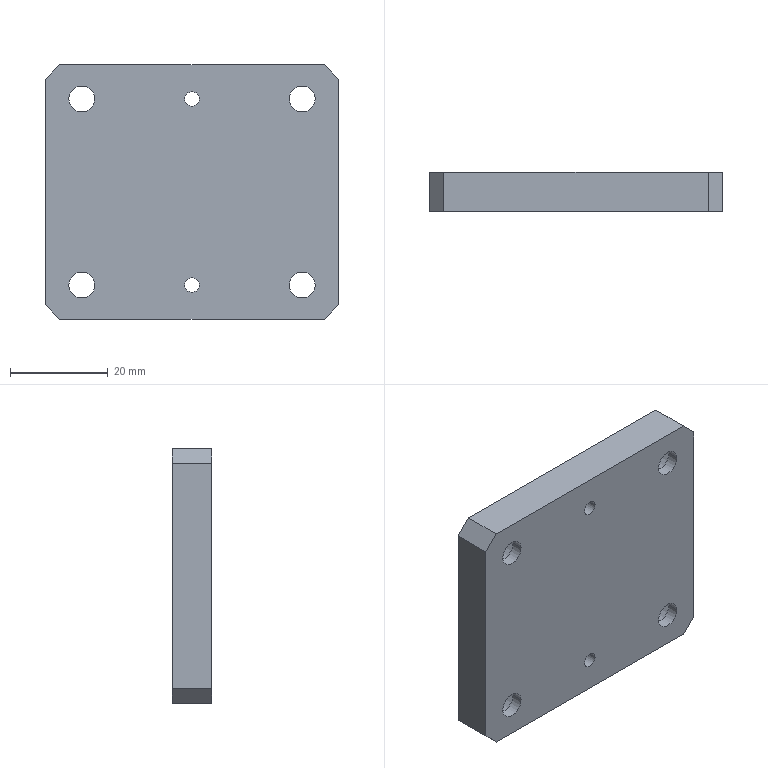Component | SolidWorks | SFTJ-08-ModuleAdapterBlock-1 | 1 solid | 34 faces | box 60 x 8 x 52 mm | volume 22709 mm3 | cylinder 20 | plane 14 | commonest cylinder face diameters 10 x8 5.3 x8 3 x4
build123d program:
from build123d import *

# Parameters (mm, degrees)
SKETCH1_W                                            = 60
SKETCH1_H                                            = 52
BOSS_EXTRUDE1_DEPTH                                  = 4
HOLE_SIZE_ACCORDING_TO_HEX_SOCKET_HEAD_C_D           = 5.3
HOLE_SIZE_ACCORDING_TO_HEX_SOCKET_HEAD_C_CBORE_D     = 10
HOLE_SIZE_ACCORDING_TO_HEX_SOCKET_HEAD_C_CBORE_DEPTH = 5.7
SIZE_MM_DOWEL_PIN_HOLE1_D                            = 3
CHAMFER1_SIZE                                        = 3


with BuildPart() as part:
    # Sketch1 → Boss-Extrude1 (new, symmetric)
    with BuildSketch(Plane.XY):
        Rectangle(SKETCH1_W, SKETCH1_H)
    extrude(amount=BOSS_EXTRUDE1_DEPTH, both=True)

    # Hole Size according to Hex Socket Head C (through all)
    with Locations(Plane.XY.offset(4)):
        with Locations((-22.5, 19), (22.5, 19), (-22.5, -19), (22.5, -19)):
            CounterBoreHole(HOLE_SIZE_ACCORDING_TO_HEX_SOCKET_HEAD_C_D / 2, HOLE_SIZE_ACCORDING_TO_HEX_SOCKET_HEAD_C_CBORE_D / 2, HOLE_SIZE_ACCORDING_TO_HEX_SOCKET_HEAD_C_CBORE_DEPTH)

    # Size mm Dowel Pin Hole1 (through all)
    with Locations(Plane(origin=(0, 0, -4), x_dir=(-1, 0, 0), z_dir=(0, 0, -1))):
        with Locations((0, -19), (0, 19)):
            Hole(SIZE_MM_DOWEL_PIN_HOLE1_D / 2)

    # Chamfer1
    chamfer1_edges = [part.edges().sort_by_distance(p)[0] for p in [
        (30, -26, 0),
        (-30, -26, 0),
        (-30, 26, 0),
        (30, 26, 0),
    ]]
    chamfer(chamfer1_edges, length=CHAMFER1_SIZE)


solid = part.part

# Placed as in the assembly
solid = solid.moved(Location((-235.009, 44.721, 38.589), (-90, 0, 0)))
STEP:
#1=COLOUR_RGB('',0.7922,0.8196,0.9333);
#2=FILL_AREA_STYLE_COLOUR('',#1);
#3=FILL_AREA_STYLE('',(#2));
#4=SURFACE_STYLE_FILL_AREA(#3);
#5=SURFACE_SIDE_STYLE('',(#4));
#6=SURFACE_STYLE_USAGE(.BOTH.,#5);
#7=PRESENTATION_STYLE_ASSIGNMENT((#6));
#8=CARTESIAN_POINT('',(-9.193,1.918,2.267));
#9=VERTEX_POINT('',#8);
#10=CARTESIAN_POINT('',(-9.311,1.918,2.267));
#11=VERTEX_POINT('',#10);
#12=CARTESIAN_POINT('',(-9.252,1.918,2.267));
#13=DIRECTION('',(0.,-1.,-0.));
#14=DIRECTION('',(-1.,0.,0.));
#15=AXIS2_PLACEMENT_3D('',#12,#13,#14);
#16=CIRCLE('',#15,0.05906);
#17=EDGE_CURVE('',#9,#11,#16,.T.);
#18=ORIENTED_EDGE('',*,*,#17,.F.);
#19=CARTESIAN_POINT('',(-9.193,1.603,2.267));
#20=VERTEX_POINT('',#19);
#21=CARTESIAN_POINT('',(-9.193,1.603,2.267));
#22=DIRECTION('',(0.,-1.,-0.));
#23=VECTOR('',#22,39.37);
#24=LINE('',#21,#23);
#25=EDGE_CURVE('',#9,#20,#24,.T.);
#26=ORIENTED_EDGE('',*,*,#25,.T.);
#27=CARTESIAN_POINT('',(-9.311,1.603,2.267));
#28=VERTEX_POINT('',#27);
#29=CARTESIAN_POINT('',(-9.252,1.603,2.267));
#30=DIRECTION('',(0.,-1.,-0.));
#31=DIRECTION('',(-1.,0.,0.));
#32=AXIS2_PLACEMENT_3D('',#29,#30,#31);
#33=CIRCLE('',#32,0.05906);
#34=EDGE_CURVE('',#20,#28,#33,.T.);
#35=ORIENTED_EDGE('',*,*,#34,.T.);
#36=CARTESIAN_POINT('',(-9.311,1.603,2.267));
#37=DIRECTION('',(0.,-1.,-0.));
#38=VECTOR('',#37,39.37);
#39=LINE('',#36,#38);
#40=EDGE_CURVE('',#11,#28,#39,.T.);
#41=ORIENTED_EDGE('',*,*,#40,.F.);
#42=EDGE_LOOP('',(#18,#26,#35,#41));
#43=FACE_OUTER_BOUND('',#42,.T.);
#44=CARTESIAN_POINT('',(-9.252,1.603,2.267));
#45=DIRECTION('',(0.,-1.,-0.));
#46=DIRECTION('',(-1.,0.,0.));
#47=AXIS2_PLACEMENT_3D('',#44,#45,#46);
#48=CYLINDRICAL_SURFACE('',#47,0.05906);
#49=ADVANCED_FACE('',(#43),#48,.F.);
#50=CARTESIAN_POINT('',(-9.193,1.918,0.7712));
#51=VERTEX_POINT('',#50);
#52=CARTESIAN_POINT('',(-9.311,1.918,0.7712));
#53=VERTEX_POINT('',#52);
#54=CARTESIAN_POINT('',(-9.252,1.918,0.7712));
#55=DIRECTION('',(0.,-1.,-0.));
#56=DIRECTION('',(-1.,0.,0.));
#57=AXIS2_PLACEMENT_3D('',#54,#55,#56);
#58=CIRCLE('',#57,0.05906);
#59=EDGE_CURVE('',#51,#53,#58,.T.);
#60=ORIENTED_EDGE('',*,*,#59,.F.);
#61=CARTESIAN_POINT('',(-9.193,1.603,0.7712));
#62=VERTEX_POINT('',#61);
#63=CARTESIAN_POINT('',(-9.193,1.603,0.7712));
#64=DIRECTION('',(0.,-1.,-0.));
#65=VECTOR('',#64,39.37);
#66=LINE('',#63,#65);
#67=EDGE_CURVE('',#51,#62,#66,.T.);
#68=ORIENTED_EDGE('',*,*,#67,.T.);
#69=CARTESIAN_POINT('',(-9.311,1.603,0.7712));
#70=VERTEX_POINT('',#69);
#71=CARTESIAN_POINT('',(-9.252,1.603,0.7712));
#72=DIRECTION('',(0.,-1.,-0.));
#73=DIRECTION('',(-1.,0.,0.));
#74=AXIS2_PLACEMENT_3D('',#71,#72,#73);
#75=CIRCLE('',#74,0.05906);
#76=EDGE_CURVE('',#62,#70,#75,.T.);
#77=ORIENTED_EDGE('',*,*,#76,.T.);
#78=CARTESIAN_POINT('',(-9.311,1.603,0.7712));
#79=DIRECTION('',(0.,-1.,-0.));
#80=VECTOR('',#79,39.37);
#81=LINE('',#78,#80);
#82=EDGE_CURVE('',#53,#70,#81,.T.);
#83=ORIENTED_EDGE('',*,*,#82,.F.);
#84=EDGE_LOOP('',(#60,#68,#77,#83));
#85=FACE_OUTER_BOUND('',#84,.T.);
#86=CARTESIAN_POINT('',(-9.252,1.603,0.7712));
#87=DIRECTION('',(0.,-1.,-0.));
#88=DIRECTION('',(-1.,0.,0.));
#89=AXIS2_PLACEMENT_3D('',#86,#87,#88);
#90=CYLINDRICAL_SURFACE('',#89,0.05906);
#91=ADVANCED_FACE('',(#85),#90,.F.);
#92=CARTESIAN_POINT('',(-10.335,1.694,0.7712));
#93=VERTEX_POINT('',#92);
#94=CARTESIAN_POINT('',(-9.941,1.694,0.7712));
#95=VERTEX_POINT('',#94);
#96=CARTESIAN_POINT('',(-10.138,1.694,0.7712));
#97=DIRECTION('',(-0.,1.,0.));
#98=DIRECTION('',(1.,0.,0.));
#99=AXIS2_PLACEMENT_3D('',#96,#97,#98);
#100=CIRCLE('',#99,0.1969);
#101=EDGE_CURVE('',#93,#95,#100,.T.);
#102=ORIENTED_EDGE('',*,*,#101,.F.);
#103=CARTESIAN_POINT('',(-10.335,1.918,0.7712));
#104=VERTEX_POINT('',#103);
#105=CARTESIAN_POINT('',(-10.335,1.918,0.7712));
#106=DIRECTION('',(-0.,1.,0.));
#107=VECTOR('',#106,39.37);
#108=LINE('',#105,#107);
#109=EDGE_CURVE('',#93,#104,#108,.T.);
#110=ORIENTED_EDGE('',*,*,#109,.T.);
#111=CARTESIAN_POINT('',(-9.941,1.918,0.7712));
#112=VERTEX_POINT('',#111);
#113=CARTESIAN_POINT('',(-10.138,1.918,0.7712));
#114=DIRECTION('',(-0.,1.,0.));
#115=DIRECTION('',(1.,0.,0.));
#116=AXIS2_PLACEMENT_3D('',#113,#114,#115);
#117=CIRCLE('',#116,0.1969);
#118=EDGE_CURVE('',#104,#112,#117,.T.);
#119=ORIENTED_EDGE('',*,*,#118,.T.);
#120=CARTESIAN_POINT('',(-9.941,1.918,0.7712));
#121=DIRECTION('',(-0.,1.,0.));
#122=VECTOR('',#121,39.37);
#123=LINE('',#120,#122);
#124=EDGE_CURVE('',#95,#112,#123,.T.);
#125=ORIENTED_EDGE('',*,*,#124,.F.);
#126=EDGE_LOOP('',(#102,#110,#119,#125));
#127=FACE_OUTER_BOUND('',#126,.T.);
#128=CARTESIAN_POINT('',(-10.138,1.918,0.7712));
#129=DIRECTION('',(-0.,1.,0.));
#130=DIRECTION('',(1.,0.,0.));
#131=AXIS2_PLACEMENT_3D('',#128,#129,#130);
#132=CYLINDRICAL_SURFACE('',#131,0.1969);
#133=ADVANCED_FACE('',(#127),#132,.F.);
#134=CARTESIAN_POINT('',(-10.242,1.603,0.7712));
#135=VERTEX_POINT('',#134);
#136=CARTESIAN_POINT('',(-10.034,1.603,0.7712));
#137=VERTEX_POINT('',#136);
#138=CARTESIAN_POINT('',(-10.138,1.603,0.7712));
#139=DIRECTION('',(-0.,1.,0.));
#140=DIRECTION('',(1.,0.,0.));
#141=AXIS2_PLACEMENT_3D('',#138,#139,#140);
#142=CIRCLE('',#141,0.1043);
#143=EDGE_CURVE('',#135,#137,#142,.T.);
#144=ORIENTED_EDGE('',*,*,#143,.F.);
#145=CARTESIAN_POINT('',(-10.242,1.694,0.7712));
#146=VERTEX_POINT('',#145);
#147=CARTESIAN_POINT('',(-10.242,1.918,0.7712));
#148=DIRECTION('',(-0.,1.,0.));
#149=VECTOR('',#148,39.37);
#150=LINE('',#147,#149);
#151=EDGE_CURVE('',#135,#146,#150,.T.);
#152=ORIENTED_EDGE('',*,*,#151,.T.);
#153=CARTESIAN_POINT('',(-10.034,1.694,0.7712));
#154=VERTEX_POINT('',#153);
#155=CARTESIAN_POINT('',(-10.138,1.694,0.7712));
#156=DIRECTION('',(-0.,1.,0.));
#157=DIRECTION('',(1.,0.,0.));
#158=AXIS2_PLACEMENT_3D('',#155,#156,#157);
#159=CIRCLE('',#158,0.1043);
#160=EDGE_CURVE('',#146,#154,#159,.T.);
#161=ORIENTED_EDGE('',*,*,#160,.T.);
#162=CARTESIAN_POINT('',(-10.034,1.918,0.7712));
#163=DIRECTION('',(-0.,1.,0.));
#164=VECTOR('',#163,39.37);
#165=LINE('',#162,#164);
#166=EDGE_CURVE('',#137,#154,#165,.T.);
#167=ORIENTED_EDGE('',*,*,#166,.F.);
#168=EDGE_LOOP('',(#144,#152,#161,#167));
#169=FACE_OUTER_BOUND('',#168,.T.);
#170=CARTESIAN_POINT('',(-10.138,1.918,0.7712));
#171=DIRECTION('',(-0.,1.,0.));
#172=DIRECTION('',(1.,0.,0.));
#173=AXIS2_PLACEMENT_3D('',#170,#171,#172);
#174=CYLINDRICAL_SURFACE('',#173,0.1043);
#175=ADVANCED_FACE('',(#169),#174,.F.);
#176=CARTESIAN_POINT('',(-8.563,1.694,0.7712));
#177=VERTEX_POINT('',#176);
#178=CARTESIAN_POINT('',(-8.17,1.694,0.7712));
#179=VERTEX_POINT('',#178);
#180=CARTESIAN_POINT('',(-8.367,1.694,0.7712));
#181=DIRECTION('',(-0.,1.,0.));
#182=DIRECTION('',(1.,0.,0.));
#183=AXIS2_PLACEMENT_3D('',#180,#181,#182);
#184=CIRCLE('',#183,0.1969);
#185=EDGE_CURVE('',#177,#179,#184,.T.);
#186=ORIENTED_EDGE('',*,*,#185,.F.);
#187=CARTESIAN_POINT('',(-8.563,1.918,0.7712));
#188=VERTEX_POINT('',#187);
#189=CARTESIAN_POINT('',(-8.563,1.918,0.7712));
#190=DIRECTION('',(-0.,1.,0.));
#191=VECTOR('',#190,39.37);
#192=LINE('',#189,#191);
#193=EDGE_CURVE('',#177,#188,#192,.T.);
#194=ORIENTED_EDGE('',*,*,#193,.T.);
#195=CARTESIAN_POINT('',(-8.17,1.918,0.7712));
#196=VERTEX_POINT('',#195);
#197=CARTESIAN_POINT('',(-8.367,1.918,0.7712));
#198=DIRECTION('',(-0.,1.,0.));
#199=DIRECTION('',(1.,0.,0.));
#200=AXIS2_PLACEMENT_3D('',#197,#198,#199);
#201=CIRCLE('',#200,0.1969);
#202=EDGE_CURVE('',#188,#196,#201,.T.);
#203=ORIENTED_EDGE('',*,*,#202,.T.);
#204=CARTESIAN_POINT('',(-8.17,1.918,0.7712));
#205=DIRECTION('',(-0.,1.,0.));
#206=VECTOR('',#205,39.37);
#207=LINE('',#204,#206);
#208=EDGE_CURVE('',#179,#196,#207,.T.);
#209=ORIENTED_EDGE('',*,*,#208,.F.);
#210=EDGE_LOOP('',(#186,#194,#203,#209));
#211=FACE_OUTER_BOUND('',#210,.T.);
#212=CARTESIAN_POINT('',(-8.367,1.918,0.7712));
#213=DIRECTION('',(-0.,1.,0.));
#214=DIRECTION('',(1.,0.,0.));
#215=AXIS2_PLACEMENT_3D('',#212,#213,#214);
#216=CYLINDRICAL_SURFACE('',#215,0.1969);
#217=ADVANCED_FACE('',(#211),#216,.F.);
#218=CARTESIAN_POINT('',(-8.471,1.603,0.7712));
#219=VERTEX_POINT('',#218);
#220=CARTESIAN_POINT('',(-8.262,1.603,0.7712));
#221=VERTEX_POINT('',#220);
#222=CARTESIAN_POINT('',(-8.367,1.603,0.7712));
#223=DIRECTION('',(-0.,1.,0.));
#224=DIRECTION('',(1.,0.,0.));
#225=AXIS2_PLACEMENT_3D('',#222,#223,#224);
#226=CIRCLE('',#225,0.1043);
#227=EDGE_CURVE('',#219,#221,#226,.T.);
#228=ORIENTED_EDGE('',*,*,#227,.F.);
#229=CARTESIAN_POINT('',(-8.471,1.694,0.7712));
#230=VERTEX_POINT('',#229);
#231=CARTESIAN_POINT('',(-8.471,1.918,0.7712));
#232=DIRECTION('',(-0.,1.,0.));
#233=VECTOR('',#232,39.37);
#234=LINE('',#231,#233);
#235=EDGE_CURVE('',#219,#230,#234,.T.);
#236=ORIENTED_EDGE('',*,*,#235,.T.);
#237=CARTESIAN_POINT('',(-8.262,1.694,0.7712));
#238=VERTEX_POINT('',#237);
#239=CARTESIAN_POINT('',(-8.367,1.694,0.7712));
#240=DIRECTION('',(-0.,1.,0.));
#241=DIRECTION('',(1.,0.,0.));
#242=AXIS2_PLACEMENT_3D('',#239,#240,#241);
#243=CIRCLE('',#242,0.1043);
#244=EDGE_CURVE('',#230,#238,#243,.T.);
#245=ORIENTED_EDGE('',*,*,#244,.T.);
#246=CARTESIAN_POINT('',(-8.262,1.918,0.7712));
#247=DIRECTION('',(-0.,1.,0.));
#248=VECTOR('',#247,39.37);
#249=LINE('',#246,#248);
#250=EDGE_CURVE('',#221,#238,#249,.T.);
#251=ORIENTED_EDGE('',*,*,#250,.F.);
#252=EDGE_LOOP('',(#228,#236,#245,#251));
#253=FACE_OUTER_BOUND('',#252,.T.);
#254=CARTESIAN_POINT('',(-8.367,1.918,0.7712));
#255=DIRECTION('',(-0.,1.,0.));
#256=DIRECTION('',(1.,0.,0.));
#257=AXIS2_PLACEMENT_3D('',#254,#255,#256);
#258=CYLINDRICAL_SURFACE('',#257,0.1043);
#259=ADVANCED_FACE('',(#253),#258,.F.);
#260=CARTESIAN_POINT('',(-10.335,1.694,2.267));
#261=VERTEX_POINT('',#260);
#262=CARTESIAN_POINT('',(-9.941,1.694,2.267));
#263=VERTEX_POINT('',#262);
#264=CARTESIAN_POINT('',(-10.138,1.694,2.267));
#265=DIRECTION('',(-0.,1.,0.));
#266=DIRECTION('',(1.,0.,0.));
#267=AXIS2_PLACEMENT_3D('',#264,#265,#266);
#268=CIRCLE('',#267,0.1969);
#269=EDGE_CURVE('',#261,#263,#268,.T.);
#270=ORIENTED_EDGE('',*,*,#269,.F.);
#271=CARTESIAN_POINT('',(-10.335,1.918,2.267));
#272=VERTEX_POINT('',#271);
#273=CARTESIAN_POINT('',(-10.335,1.918,2.267));
#274=DIRECTION('',(-0.,1.,0.));
#275=VECTOR('',#274,39.37);
#276=LINE('',#273,#275);
#277=EDGE_CURVE('',#261,#272,#276,.T.);
#278=ORIENTED_EDGE('',*,*,#277,.T.);
#279=CARTESIAN_POINT('',(-9.941,1.918,2.267));
#280=VERTEX_POINT('',#279);
#281=CARTESIAN_POINT('',(-10.138,1.918,2.267));
#282=DIRECTION('',(-0.,1.,0.));
#283=DIRECTION('',(1.,0.,0.));
#284=AXIS2_PLACEMENT_3D('',#281,#282,#283);
#285=CIRCLE('',#284,0.1969);
#286=EDGE_CURVE('',#272,#280,#285,.T.);
#287=ORIENTED_EDGE('',*,*,#286,.T.);
#288=CARTESIAN_POINT('',(-9.941,1.918,2.267));
#289=DIRECTION('',(-0.,1.,0.));
#290=VECTOR('',#289,39.37);
#291=LINE('',#288,#290);
#292=EDGE_CURVE('',#263,#280,#291,.T.);
#293=ORIENTED_EDGE('',*,*,#292,.F.);
#294=EDGE_LOOP('',(#270,#278,#287,#293));
#295=FACE_OUTER_BOUND('',#294,.T.);
#296=CARTESIAN_POINT('',(-10.138,1.918,2.267));
#297=DIRECTION('',(-0.,1.,0.));
#298=DIRECTION('',(1.,0.,0.));
#299=AXIS2_PLACEMENT_3D('',#296,#297,#298);
#300=CYLINDRICAL_SURFACE('',#299,0.1969);
#301=ADVANCED_FACE('',(#295),#300,.F.);
#302=CARTESIAN_POINT('',(-10.242,1.603,2.267));
#303=VERTEX_POINT('',#302);
#304=CARTESIAN_POINT('',(-10.034,1.603,2.267));
#305=VERTEX_POINT('',#304);
#306=CARTESIAN_POINT('',(-10.138,1.603,2.267));
#307=DIRECTION('',(-0.,1.,0.));
#308=DIRECTION('',(1.,0.,0.));
#309=AXIS2_PLACEMENT_3D('',#306,#307,#308);
#310=CIRCLE('',#309,0.1043);
#311=EDGE_CURVE('',#303,#305,#310,.T.);
#312=ORIENTED_EDGE('',*,*,#311,.F.);
#313=CARTESIAN_POINT('',(-10.242,1.694,2.267));
#314=VERTEX_POINT('',#313);
#315=CARTESIAN_POINT('',(-10.242,1.918,2.267));
#316=DIRECTION('',(-0.,1.,0.));
#317=VECTOR('',#316,39.37);
#318=LINE('',#315,#317);
#319=EDGE_CURVE('',#303,#314,#318,.T.);
#320=ORIENTED_EDGE('',*,*,#319,.T.);
#321=CARTESIAN_POINT('',(-10.034,1.694,2.267));
#322=VERTEX_POINT('',#321);
#323=CARTESIAN_POINT('',(-10.138,1.694,2.267));
#324=DIRECTION('',(-0.,1.,0.));
#325=DIRECTION('',(1.,0.,0.));
#326=AXIS2_PLACEMENT_3D('',#323,#324,#325);
#327=CIRCLE('',#326,0.1043);
#328=EDGE_CURVE('',#314,#322,#327,.T.);
#329=ORIENTED_EDGE('',*,*,#328,.T.);
#330=CARTESIAN_POINT('',(-10.034,1.918,2.267));
#331=DIRECTION('',(-0.,1.,0.));
#332=VECTOR('',#331,39.37);
#333=LINE('',#330,#332);
#334=EDGE_CURVE('',#305,#322,#333,.T.);
#335=ORIENTED_EDGE('',*,*,#334,.F.);
#336=EDGE_LOOP('',(#312,#320,#329,#335));
#337=FACE_OUTER_BOUND('',#336,.T.);
#338=CARTESIAN_POINT('',(-10.138,1.918,2.267));
#339=DIRECTION('',(-0.,1.,0.));
#340=DIRECTION('',(1.,0.,0.));
#341=AXIS2_PLACEMENT_3D('',#338,#339,#340);
#342=CYLINDRICAL_SURFACE('',#341,0.1043);
#343=ADVANCED_FACE('',(#337),#342,.F.);
#344=CARTESIAN_POINT('',(-8.563,1.694,2.267));
#345=VERTEX_POINT('',#344);
#346=CARTESIAN_POINT('',(-8.17,1.694,2.267));
#347=VERTEX_POINT('',#346);
#348=CARTESIAN_POINT('',(-8.367,1.694,2.267));
#349=DIRECTION('',(-0.,1.,0.));
#350=DIRECTION('',(1.,0.,0.));
#351=AXIS2_PLACEMENT_3D('',#348,#349,#350);
#352=CIRCLE('',#351,0.1969);
#353=EDGE_CURVE('',#345,#347,#352,.T.);
#354=ORIENTED_EDGE('',*,*,#353,.F.);
#355=CARTESIAN_POINT('',(-8.563,1.918,2.267));
#356=VERTEX_POINT('',#355);
#357=CARTESIAN_POINT('',(-8.563,1.918,2.267));
#358=DIRECTION('',(-0.,1.,0.));
#359=VECTOR('',#358,39.37);
#360=LINE('',#357,#359);
#361=EDGE_CURVE('',#345,#356,#360,.T.);
#362=ORIENTED_EDGE('',*,*,#361,.T.);
#363=CARTESIAN_POINT('',(-8.17,1.918,2.267));
#364=VERTEX_POINT('',#363);
#365=CARTESIAN_POINT('',(-8.367,1.918,2.267));
#366=DIRECTION('',(-0.,1.,0.));
#367=DIRECTION('',(1.,0.,0.));
#368=AXIS2_PLACEMENT_3D('',#365,#366,#367);
#369=CIRCLE('',#368,0.1969);
#370=EDGE_CURVE('',#356,#364,#369,.T.);
#371=ORIENTED_EDGE('',*,*,#370,.T.);
#372=CARTESIAN_POINT('',(-8.17,1.918,2.267));
#373=DIRECTION('',(-0.,1.,0.));
#374=VECTOR('',#373,39.37);
#375=LINE('',#372,#374);
#376=EDGE_CURVE('',#347,#364,#375,.T.);
#377=ORIENTED_EDGE('',*,*,#376,.F.);
#378=EDGE_LOOP('',(#354,#362,#371,#377));
#379=FACE_OUTER_BOUND('',#378,.T.);
#380=CARTESIAN_POINT('',(-8.367,1.918,2.267));
#381=DIRECTION('',(-0.,1.,0.));
#382=DIRECTION('',(1.,0.,0.));
#383=AXIS2_PLACEMENT_3D('',#380,#381,#382);
#384=CYLINDRICAL_SURFACE('',#383,0.1969);
#385=ADVANCED_FACE('',(#379),#384,.F.);
#386=CARTESIAN_POINT('',(-8.471,1.603,2.267));
#387=VERTEX_POINT('',#386);
#388=CARTESIAN_POINT('',(-8.262,1.603,2.267));
#389=VERTEX_POINT('',#388);
#390=CARTESIAN_POINT('',(-8.367,1.603,2.267));
#391=DIRECTION('',(-0.,1.,0.));
#392=DIRECTION('',(1.,0.,0.));
#393=AXIS2_PLACEMENT_3D('',#390,#391,#392);
#394=CIRCLE('',#393,0.1043);
#395=EDGE_CURVE('',#387,#389,#394,.T.);
#396=ORIENTED_EDGE('',*,*,#395,.F.);
#397=CARTESIAN_POINT('',(-8.471,1.694,2.267));
#398=VERTEX_POINT('',#397);
#399=CARTESIAN_POINT('',(-8.471,1.918,2.267));
#400=DIRECTION('',(-0.,1.,0.));
#401=VECTOR('',#400,39.37);
#402=LINE('',#399,#401);
#403=EDGE_CURVE('',#387,#398,#402,.T.);
#404=ORIENTED_EDGE('',*,*,#403,.T.);
#405=CARTESIAN_POINT('',(-8.262,1.694,2.267));
#406=VERTEX_POINT('',#405);
#407=CARTESIAN_POINT('',(-8.367,1.694,2.267));
#408=DIRECTION('',(-0.,1.,0.));
#409=DIRECTION('',(1.,0.,0.));
#410=AXIS2_PLACEMENT_3D('',#407,#408,#409);
#411=CIRCLE('',#410,0.1043);
#412=EDGE_CURVE('',#398,#406,#411,.T.);
#413=ORIENTED_EDGE('',*,*,#412,.T.);
#414=CARTESIAN_POINT('',(-8.262,1.918,2.267));
#415=DIRECTION('',(-0.,1.,0.));
#416=VECTOR('',#415,39.37);
#417=LINE('',#414,#416);
#418=EDGE_CURVE('',#389,#406,#417,.T.);
#419=ORIENTED_EDGE('',*,*,#418,.F.);
#420=EDGE_LOOP('',(#396,#404,#413,#419));
#421=FACE_OUTER_BOUND('',#420,.T.);
#422=CARTESIAN_POINT('',(-8.367,1.918,2.267));
#423=DIRECTION('',(-0.,1.,0.));
#424=DIRECTION('',(1.,0.,0.));
#425=AXIS2_PLACEMENT_3D('',#422,#423,#424);
#426=CYLINDRICAL_SURFACE('',#425,0.1043);
#427=ADVANCED_FACE('',(#421),#426,.F.);
#428=CARTESIAN_POINT('',(-8.071,1.918,2.425));
#429=VERTEX_POINT('',#428);
#430=CARTESIAN_POINT('',(-8.071,1.918,0.6137));
#431=VERTEX_POINT('',#430);
#432=CARTESIAN_POINT('',(-8.071,1.918,0.4956));
#433=DIRECTION('',(-0.,0.,-1.));
#434=VECTOR('',#433,39.37);
#435=LINE('',#432,#434);
#436=EDGE_CURVE('',#429,#431,#435,.T.);
#437=ORIENTED_EDGE('',*,*,#436,.F.);
#438=CARTESIAN_POINT('',(-8.071,1.603,2.425));
#439=VERTEX_POINT('',#438);
#440=CARTESIAN_POINT('',(-8.071,1.918,2.425));
#441=DIRECTION('',(0.,-1.,-0.));
#442=VECTOR('',#441,39.37);
#443=LINE('',#440,#442);
#444=EDGE_CURVE('',#429,#439,#443,.T.);
#445=ORIENTED_EDGE('',*,*,#444,.T.);
#446=CARTESIAN_POINT('',(-8.071,1.603,0.6137));
#447=VERTEX_POINT('',#446);
#448=CARTESIAN_POINT('',(-8.071,1.603,0.4956));
#449=DIRECTION('',(-0.,0.,-1.));
#450=VECTOR('',#449,39.37);
#451=LINE('',#448,#450);
#452=EDGE_CURVE('',#439,#447,#451,.T.);
#453=ORIENTED_EDGE('',*,*,#452,.T.);
#454=CARTESIAN_POINT('',(-8.071,1.918,0.6137));
#455=DIRECTION('',(-0.,1.,0.));
#456=VECTOR('',#455,39.37);
#457=LINE('',#454,#456);
#458=EDGE_CURVE('',#447,#431,#457,.T.);
#459=ORIENTED_EDGE('',*,*,#458,.T.);
#460=EDGE_LOOP('',(#437,#445,#453,#459));
#461=FACE_OUTER_BOUND('',#460,.T.);
#462=CARTESIAN_POINT('',(-8.071,1.918,0.4956));
#463=DIRECTION('',(-1.,-0.,0.));
#464=DIRECTION('',(0.,-0.,1.));
#465=AXIS2_PLACEMENT_3D('',#462,#463,#464);
#466=PLANE('',#465);
#467=ADVANCED_FACE('',(#461),#466,.F.);
#468=CARTESIAN_POINT('',(-8.189,1.918,0.4956));
#469=VERTEX_POINT('',#468);
#470=CARTESIAN_POINT('',(-10.315,1.918,0.4956));
#471=VERTEX_POINT('',#470);
#472=CARTESIAN_POINT('',(-10.433,1.918,0.4956));
#473=DIRECTION('',(-1.,-0.,-0.));
#474=VECTOR('',#473,39.37);
#475=LINE('',#472,#474);
#476=EDGE_CURVE('',#469,#471,#475,.T.);
#477=ORIENTED_EDGE('',*,*,#476,.F.);
#478=CARTESIAN_POINT('',(-8.189,1.603,0.4956));
#479=VERTEX_POINT('',#478);
#480=CARTESIAN_POINT('',(-8.189,1.918,0.4956));
#481=DIRECTION('',(0.,-1.,-0.));
#482=VECTOR('',#481,39.37);
#483=LINE('',#480,#482);
#484=EDGE_CURVE('',#469,#479,#483,.T.);
#485=ORIENTED_EDGE('',*,*,#484,.T.);
#486=CARTESIAN_POINT('',(-10.315,1.603,0.4956));
#487=VERTEX_POINT('',#486);
#488=CARTESIAN_POINT('',(-10.433,1.603,0.4956));
#489=DIRECTION('',(-1.,-0.,-0.));
#490=VECTOR('',#489,39.37);
#491=LINE('',#488,#490);
#492=EDGE_CURVE('',#479,#487,#491,.T.);
#493=ORIENTED_EDGE('',*,*,#492,.T.);
#494=CARTESIAN_POINT('',(-10.315,1.918,0.4956));
#495=DIRECTION('',(-0.,1.,0.));
#496=VECTOR('',#495,39.37);
#497=LINE('',#494,#496);
#498=EDGE_CURVE('',#487,#471,#497,.T.);
#499=ORIENTED_EDGE('',*,*,#498,.T.);
#500=EDGE_LOOP('',(#477,#485,#493,#499));
#501=FACE_OUTER_BOUND('',#500,.T.);
#502=CARTESIAN_POINT('',(-10.433,1.918,0.4956));
#503=DIRECTION('',(-0.,-0.,1.));
#504=DIRECTION('',(0.,-1.,-0.));
#505=AXIS2_PLACEMENT_3D('',#502,#503,#504);
#506=PLANE('',#505);
#507=ADVANCED_FACE('',(#501),#506,.F.);
#508=CARTESIAN_POINT('',(-10.433,1.603,0.6137));
#509=VERTEX_POINT('',#508);
#510=CARTESIAN_POINT('',(-10.433,1.603,2.425));
#511=VERTEX_POINT('',#510);
#512=CARTESIAN_POINT('',(-10.433,1.603,0.4956));
#513=DIRECTION('',(0.,-0.,1.));
#514=VECTOR('',#513,39.37);
#515=LINE('',#512,#514);
#516=EDGE_CURVE('',#509,#511,#515,.T.);
#517=ORIENTED_EDGE('',*,*,#516,.T.);
#518=CARTESIAN_POINT('',(-10.433,1.918,2.425));
#519=VERTEX_POINT('',#518);
#520=CARTESIAN_POINT('',(-10.433,1.918,2.425));
#521=DIRECTION('',(-0.,1.,0.));
#522=VECTOR('',#521,39.37);
#523=LINE('',#520,#522);
#524=EDGE_CURVE('',#511,#519,#523,.T.);
#525=ORIENTED_EDGE('',*,*,#524,.T.);
#526=CARTESIAN_POINT('',(-10.433,1.918,0.6137));
#527=VERTEX_POINT('',#526);
#528=CARTESIAN_POINT('',(-10.433,1.918,0.4956));
#529=DIRECTION('',(0.,-0.,1.));
#530=VECTOR('',#529,39.37);
#531=LINE('',#528,#530);
#532=EDGE_CURVE('',#527,#519,#531,.T.);
#533=ORIENTED_EDGE('',*,*,#532,.F.);
#534=CARTESIAN_POINT('',(-10.433,1.918,0.6137));
#535=DIRECTION('',(0.,-1.,-0.));
#536=VECTOR('',#535,39.37);
#537=LINE('',#534,#536);
#538=EDGE_CURVE('',#527,#509,#537,.T.);
#539=ORIENTED_EDGE('',*,*,#538,.T.);
#540=EDGE_LOOP('',(#517,#525,#533,#539));
#541=FACE_OUTER_BOUND('',#540,.T.);
#542=CARTESIAN_POINT('',(-10.433,1.918,0.4956));
#543=DIRECTION('',(1.,0.,-0.));
#544=DIRECTION('',(-0.,0.,-1.));
#545=AXIS2_PLACEMENT_3D('',#542,#543,#544);
#546=PLANE('',#545);
#547=ADVANCED_FACE('',(#541),#546,.F.);
#548=CARTESIAN_POINT('',(-10.315,1.603,2.543));
#549=VERTEX_POINT('',#548);
#550=CARTESIAN_POINT('',(-8.189,1.603,2.543));
#551=VERTEX_POINT('',#550);
#552=CARTESIAN_POINT('',(-10.433,1.603,2.543));
#553=DIRECTION('',(1.,0.,0.));
#554=VECTOR('',#553,39.37);
#555=LINE('',#552,#554);
#556=EDGE_CURVE('',#549,#551,#555,.T.);
#557=ORIENTED_EDGE('',*,*,#556,.T.);
#558=CARTESIAN_POINT('',(-8.189,1.918,2.543));
#559=VERTEX_POINT('',#558);
#560=CARTESIAN_POINT('',(-8.189,1.918,2.543));
#561=DIRECTION('',(-0.,1.,0.));
#562=VECTOR('',#561,39.37);
#563=LINE('',#560,#562);
#564=EDGE_CURVE('',#551,#559,#563,.T.);
#565=ORIENTED_EDGE('',*,*,#564,.T.);
#566=CARTESIAN_POINT('',(-10.315,1.918,2.543));
#567=VERTEX_POINT('',#566);
#568=CARTESIAN_POINT('',(-10.433,1.918,2.543));
#569=DIRECTION('',(1.,0.,0.));
#570=VECTOR('',#569,39.37);
#571=LINE('',#568,#570);
#572=EDGE_CURVE('',#567,#559,#571,.T.);
#573=ORIENTED_EDGE('',*,*,#572,.F.);
#574=CARTESIAN_POINT('',(-10.315,1.918,2.543));
#575=DIRECTION('',(0.,-1.,-0.));
#576=VECTOR('',#575,39.37);
#577=LINE('',#574,#576);
#578=EDGE_CURVE('',#567,#549,#577,.T.);
#579=ORIENTED_EDGE('',*,*,#578,.T.);
#580=EDGE_LOOP('',(#557,#565,#573,#579));
#581=FACE_OUTER_BOUND('',#580,.T.);
#582=CARTESIAN_POINT('',(-10.433,1.918,2.543));
#583=DIRECTION('',(0.,0.,-1.));
#584=DIRECTION('',(-0.,1.,0.));
#585=AXIS2_PLACEMENT_3D('',#582,#583,#584);
#586=PLANE('',#585);
#587=ADVANCED_FACE('',(#581),#586,.F.);
#588=CARTESIAN_POINT('',(-9.252,1.918,2.267));
#589=DIRECTION('',(0.,-1.,-0.));
#590=DIRECTION('',(-1.,0.,0.));
#591=AXIS2_PLACEMENT_3D('',#588,#589,#590);
#592=CIRCLE('',#591,0.05906);
#593=EDGE_CURVE('',#11,#9,#592,.T.);
#594=ORIENTED_EDGE('',*,*,#593,.T.);
#595=ORIENTED_EDGE('',*,*,#17,.T.);
#596=EDGE_LOOP('',(#594,#595));
#597=FACE_BOUND('',#596,.T.);
#598=CARTESIAN_POINT('',(-9.252,1.918,0.7712));
#599=DIRECTION('',(0.,-1.,-0.));
#600=DIRECTION('',(-1.,0.,0.));
#601=AXIS2_PLACEMENT_3D('',#598,#599,#600);
#602=CIRCLE('',#601,0.05906);
#603=EDGE_CURVE('',#53,#51,#602,.T.);
#604=ORIENTED_EDGE('',*,*,#603,.T.);
#605=ORIENTED_EDGE('',*,*,#59,.T.);
#606=EDGE_LOOP('',(#604,#605));
#607=FACE_BOUND('',#606,.T.);
#608=CARTESIAN_POINT('',(-10.138,1.918,0.7712));
#609=DIRECTION('',(-0.,1.,0.));
#610=DIRECTION('',(1.,0.,0.));
#611=AXIS2_PLACEMENT_3D('',#608,#609,#610);
#612=CIRCLE('',#611,0.1969);
#613=EDGE_CURVE('',#112,#104,#612,.T.);
#614=ORIENTED_EDGE('',*,*,#613,.F.);
#615=ORIENTED_EDGE('',*,*,#118,.F.);
#616=EDGE_LOOP('',(#614,#615));
#617=FACE_BOUND('',#616,.T.);
#618=CARTESIAN_POINT('',(-8.367,1.918,0.7712));
#619=DIRECTION('',(-0.,1.,0.));
#620=DIRECTION('',(1.,0.,0.));
#621=AXIS2_PLACEMENT_3D('',#618,#619,#620);
#622=CIRCLE('',#621,0.1969);
#623=EDGE_CURVE('',#196,#188,#622,.T.);
#624=ORIENTED_EDGE('',*,*,#623,.F.);
#625=ORIENTED_EDGE('',*,*,#202,.F.);
#626=EDGE_LOOP('',(#624,#625));
#627=FACE_BOUND('',#626,.T.);
#628=CARTESIAN_POINT('',(-10.138,1.918,2.267));
#629=DIRECTION('',(-0.,1.,0.));
#630=DIRECTION('',(1.,0.,0.));
#631=AXIS2_PLACEMENT_3D('',#628,#629,#630);
#632=CIRCLE('',#631,0.1969);
#633=EDGE_CURVE('',#280,#272,#632,.T.);
#634=ORIENTED_EDGE('',*,*,#633,.F.);
#635=ORIENTED_EDGE('',*,*,#286,.F.);
#636=EDGE_LOOP('',(#634,#635));
#637=FACE_BOUND('',#636,.T.);
#638=CARTESIAN_POINT('',(-8.367,1.918,2.267));
#639=DIRECTION('',(-0.,1.,0.));
#640=DIRECTION('',(1.,0.,0.));
#641=AXIS2_PLACEMENT_3D('',#638,#639,#640);
#642=CIRCLE('',#641,0.1969);
#643=EDGE_CURVE('',#364,#356,#642,.T.);
#644=ORIENTED_EDGE('',*,*,#643,.F.);
#645=ORIENTED_EDGE('',*,*,#370,.F.);
#646=EDGE_LOOP('',(#644,#645));
#647=FACE_BOUND('',#646,.T.);
#648=ORIENTED_EDGE('',*,*,#572,.T.);
#649=CARTESIAN_POINT('',(-8.209,1.918,2.563));
#650=DIRECTION('',(0.7071,0.,-0.7071));
#651=VECTOR('',#650,39.37);
#652=LINE('',#649,#651);
#653=EDGE_CURVE('',#559,#429,#652,.T.);
#654=ORIENTED_EDGE('',*,*,#653,.T.);
#655=ORIENTED_EDGE('',*,*,#436,.T.);
#656=CARTESIAN_POINT('',(-8.209,1.918,0.4759));
#657=DIRECTION('',(-0.7071,-0.,-0.7071));
#658=VECTOR('',#657,39.37);
#659=LINE('',#656,#658);
#660=EDGE_CURVE('',#431,#469,#659,.T.);
#661=ORIENTED_EDGE('',*,*,#660,.T.);
#662=ORIENTED_EDGE('',*,*,#476,.T.);
#663=CARTESIAN_POINT('',(-10.296,1.918,0.4759));
#664=DIRECTION('',(-0.7071,-0.,0.7071));
#665=VECTOR('',#664,39.37);
#666=LINE('',#663,#665);
#667=EDGE_CURVE('',#471,#527,#666,.T.);
#668=ORIENTED_EDGE('',*,*,#667,.T.);
#669=ORIENTED_EDGE('',*,*,#532,.T.);
#670=CARTESIAN_POINT('',(-10.296,1.918,2.563));
#671=DIRECTION('',(0.7071,0.,0.7071));
#672=VECTOR('',#671,39.37);
#673=LINE('',#670,#672);
#674=EDGE_CURVE('',#519,#567,#673,.T.);
#675=ORIENTED_EDGE('',*,*,#674,.T.);
#676=EDGE_LOOP('',(#648,#654,#655,#661,#662,#668,#669,#675));
#677=FACE_OUTER_BOUND('',#676,.T.);
#678=CARTESIAN_POINT('',(-9.252,1.918,1.519));
#679=DIRECTION('',(-0.,1.,0.));
#680=DIRECTION('',(1.,0.,0.));
#681=AXIS2_PLACEMENT_3D('',#678,#679,#680);
#682=PLANE('',#681);
#683=ADVANCED_FACE('',(#597,#607,#617,#627,#637,#647,#677),#682,.T.);
#684=CARTESIAN_POINT('',(-9.252,1.603,2.267));
#685=DIRECTION('',(0.,-1.,-0.));
#686=DIRECTION('',(-1.,0.,0.));
#687=AXIS2_PLACEMENT_3D('',#684,#685,#686);
#688=CIRCLE('',#687,0.05906);
#689=EDGE_CURVE('',#28,#20,#688,.T.);
#690=ORIENTED_EDGE('',*,*,#689,.F.);
#691=ORIENTED_EDGE('',*,*,#34,.F.);
#692=EDGE_LOOP('',(#690,#691));
#693=FACE_BOUND('',#692,.T.);
#694=CARTESIAN_POINT('',(-9.252,1.603,0.7712));
#695=DIRECTION('',(0.,-1.,-0.));
#696=DIRECTION('',(-1.,0.,0.));
#697=AXIS2_PLACEMENT_3D('',#694,#695,#696);
#698=CIRCLE('',#697,0.05906);
#699=EDGE_CURVE('',#70,#62,#698,.T.);
#700=ORIENTED_EDGE('',*,*,#699,.F.);
#701=ORIENTED_EDGE('',*,*,#76,.F.);
#702=EDGE_LOOP('',(#700,#701));
#703=FACE_BOUND('',#702,.T.);
#704=CARTESIAN_POINT('',(-10.138,1.603,0.7712));
#705=DIRECTION('',(-0.,1.,0.));
#706=DIRECTION('',(1.,0.,0.));
#707=AXIS2_PLACEMENT_3D('',#704,#705,#706);
#708=CIRCLE('',#707,0.1043);
#709=EDGE_CURVE('',#137,#135,#708,.T.);
#710=ORIENTED_EDGE('',*,*,#709,.T.);
#711=ORIENTED_EDGE('',*,*,#143,.T.);
#712=EDGE_LOOP('',(#710,#711));
#713=FACE_BOUND('',#712,.T.);
#714=CARTESIAN_POINT('',(-8.367,1.603,0.7712));
#715=DIRECTION('',(-0.,1.,0.));
#716=DIRECTION('',(1.,0.,0.));
#717=AXIS2_PLACEMENT_3D('',#714,#715,#716);
#718=CIRCLE('',#717,0.1043);
#719=EDGE_CURVE('',#221,#219,#718,.T.);
#720=ORIENTED_EDGE('',*,*,#719,.T.);
#721=ORIENTED_EDGE('',*,*,#227,.T.);
#722=EDGE_LOOP('',(#720,#721));
#723=FACE_BOUND('',#722,.T.);
#724=CARTESIAN_POINT('',(-10.138,1.603,2.267));
#725=DIRECTION('',(-0.,1.,0.));
#726=DIRECTION('',(1.,0.,0.));
#727=AXIS2_PLACEMENT_3D('',#724,#725,#726);
#728=CIRCLE('',#727,0.1043);
#729=EDGE_CURVE('',#305,#303,#728,.T.);
#730=ORIENTED_EDGE('',*,*,#729,.T.);
#731=ORIENTED_EDGE('',*,*,#311,.T.);
#732=EDGE_LOOP('',(#730,#731));
#733=FACE_BOUND('',#732,.T.);
#734=CARTESIAN_POINT('',(-8.367,1.603,2.267));
#735=DIRECTION('',(-0.,1.,0.));
#736=DIRECTION('',(1.,0.,0.));
#737=AXIS2_PLACEMENT_3D('',#734,#735,#736);
#738=CIRCLE('',#737,0.1043);
#739=EDGE_CURVE('',#389,#387,#738,.T.);
#740=ORIENTED_EDGE('',*,*,#739,.T.);
#741=ORIENTED_EDGE('',*,*,#395,.T.);
#742=EDGE_LOOP('',(#740,#741));
#743=FACE_BOUND('',#742,.T.);
#744=ORIENTED_EDGE('',*,*,#452,.F.);
#745=CARTESIAN_POINT('',(-8.071,1.603,2.425));
#746=DIRECTION('',(-0.7071,-0.,0.7071));
#747=VECTOR('',#746,39.37);
#748=LINE('',#745,#747);
#749=EDGE_CURVE('',#439,#551,#748,.T.);
#750=ORIENTED_EDGE('',*,*,#749,.T.);
#751=ORIENTED_EDGE('',*,*,#556,.F.);
#752=CARTESIAN_POINT('',(-10.315,1.603,2.543));
#753=DIRECTION('',(-0.7071,-0.,-0.7071));
#754=VECTOR('',#753,39.37);
#755=LINE('',#752,#754);
#756=EDGE_CURVE('',#549,#511,#755,.T.);
#757=ORIENTED_EDGE('',*,*,#756,.T.);
#758=ORIENTED_EDGE('',*,*,#516,.F.);
#759=CARTESIAN_POINT('',(-10.433,1.603,0.6137));
#760=DIRECTION('',(0.7071,0.,-0.7071));
#761=VECTOR('',#760,39.37);
#762=LINE('',#759,#761);
#763=EDGE_CURVE('',#509,#487,#762,.T.);
#764=ORIENTED_EDGE('',*,*,#763,.T.);
#765=ORIENTED_EDGE('',*,*,#492,.F.);
#766=CARTESIAN_POINT('',(-8.189,1.603,0.4956));
#767=DIRECTION('',(0.7071,0.,0.7071));
#768=VECTOR('',#767,39.37);
#769=LINE('',#766,#768);
#770=EDGE_CURVE('',#479,#447,#769,.T.);
#771=ORIENTED_EDGE('',*,*,#770,.T.);
#772=EDGE_LOOP('',(#744,#750,#751,#757,#758,#764,#765,#771));
#773=FACE_OUTER_BOUND('',#772,.T.);
#774=CARTESIAN_POINT('',(-9.252,1.603,1.519));
#775=DIRECTION('',(-0.,1.,0.));
#776=DIRECTION('',(1.,0.,0.));
#777=AXIS2_PLACEMENT_3D('',#774,#775,#776);
#778=PLANE('',#777);
#779=ADVANCED_FACE('',(#693,#703,#713,#723,#733,#743,#773),#778,.F.);
#780=ORIENTED_EDGE('',*,*,#403,.F.);
#781=ORIENTED_EDGE('',*,*,#739,.F.);
#782=ORIENTED_EDGE('',*,*,#418,.T.);
#783=CARTESIAN_POINT('',(-8.367,1.694,2.267));
#784=DIRECTION('',(-0.,1.,0.));
#785=DIRECTION('',(1.,0.,0.));
#786=AXIS2_PLACEMENT_3D('',#783,#784,#785);
#787=CIRCLE('',#786,0.1043);
#788=EDGE_CURVE('',#406,#398,#787,.T.);
#789=ORIENTED_EDGE('',*,*,#788,.T.);
#790=EDGE_LOOP('',(#780,#781,#782,#789));
#791=FACE_OUTER_BOUND('',#790,.T.);
#792=CARTESIAN_POINT('',(-8.367,1.918,2.267));
#793=DIRECTION('',(-0.,1.,0.));
#794=DIRECTION('',(1.,0.,0.));
#795=AXIS2_PLACEMENT_3D('',#792,#793,#794);
#796=CYLINDRICAL_SURFACE('',#795,0.1043);
#797=ADVANCED_FACE('',(#791),#796,.F.);
#798=ORIENTED_EDGE('',*,*,#788,.F.);
#799=ORIENTED_EDGE('',*,*,#412,.F.);
#800=EDGE_LOOP('',(#798,#799));
#801=FACE_BOUND('',#800,.T.);
#802=CARTESIAN_POINT('',(-8.367,1.694,2.267));
#803=DIRECTION('',(-0.,1.,0.));
#804=DIRECTION('',(1.,0.,0.));
#805=AXIS2_PLACEMENT_3D('',#802,#803,#804);
#806=CIRCLE('',#805,0.1969);
#807=EDGE_CURVE('',#347,#345,#806,.T.);
#808=ORIENTED_EDGE('',*,*,#807,.T.);
#809=ORIENTED_EDGE('',*,*,#353,.T.);
#810=EDGE_LOOP('',(#808,#809));
#811=FACE_OUTER_BOUND('',#810,.T.);
#812=CARTESIAN_POINT('',(-8.262,1.694,2.267));
#813=DIRECTION('',(0.,-1.,-0.));
#814=DIRECTION('',(-1.,-0.,-0.));
#815=AXIS2_PLACEMENT_3D('',#812,#813,#814);
#816=PLANE('',#815);
#817=ADVANCED_FACE('',(#801,#811),#816,.F.);
#818=ORIENTED_EDGE('',*,*,#361,.F.);
#819=ORIENTED_EDGE('',*,*,#807,.F.);
#820=ORIENTED_EDGE('',*,*,#376,.T.);
#821=ORIENTED_EDGE('',*,*,#643,.T.);
#822=EDGE_LOOP('',(#818,#819,#820,#821));
#823=FACE_OUTER_BOUND('',#822,.T.);
#824=CARTESIAN_POINT('',(-8.367,1.918,2.267));
#825=DIRECTION('',(-0.,1.,0.));
#826=DIRECTION('',(1.,0.,0.));
#827=AXIS2_PLACEMENT_3D('',#824,#825,#826);
#828=CYLINDRICAL_SURFACE('',#827,0.1969);
#829=ADVANCED_FACE('',(#823),#828,.F.);
#830=ORIENTED_EDGE('',*,*,#319,.F.);
#831=ORIENTED_EDGE('',*,*,#729,.F.);
#832=ORIENTED_EDGE('',*,*,#334,.T.);
#833=CARTESIAN_POINT('',(-10.138,1.694,2.267));
#834=DIRECTION('',(-0.,1.,0.));
#835=DIRECTION('',(1.,0.,0.));
#836=AXIS2_PLACEMENT_3D('',#833,#834,#835);
#837=CIRCLE('',#836,0.1043);
#838=EDGE_CURVE('',#322,#314,#837,.T.);
#839=ORIENTED_EDGE('',*,*,#838,.T.);
#840=EDGE_LOOP('',(#830,#831,#832,#839));
#841=FACE_OUTER_BOUND('',#840,.T.);
#842=CARTESIAN_POINT('',(-10.138,1.918,2.267));
#843=DIRECTION('',(-0.,1.,0.));
#844=DIRECTION('',(1.,0.,0.));
#845=AXIS2_PLACEMENT_3D('',#842,#843,#844);
#846=CYLINDRICAL_SURFACE('',#845,0.1043);
#847=ADVANCED_FACE('',(#841),#846,.F.);
#848=ORIENTED_EDGE('',*,*,#838,.F.);
#849=ORIENTED_EDGE('',*,*,#328,.F.);
#850=EDGE_LOOP('',(#848,#849));
#851=FACE_BOUND('',#850,.T.);
#852=CARTESIAN_POINT('',(-10.138,1.694,2.267));
#853=DIRECTION('',(-0.,1.,0.));
#854=DIRECTION('',(1.,0.,0.));
#855=AXIS2_PLACEMENT_3D('',#852,#853,#854);
#856=CIRCLE('',#855,0.1969);
#857=EDGE_CURVE('',#263,#261,#856,.T.);
#858=ORIENTED_EDGE('',*,*,#857,.T.);
#859=ORIENTED_EDGE('',*,*,#269,.T.);
#860=EDGE_LOOP('',(#858,#859));
#861=FACE_OUTER_BOUND('',#860,.T.);
#862=CARTESIAN_POINT('',(-10.034,1.694,2.267));
#863=DIRECTION('',(0.,-1.,-0.));
#864=DIRECTION('',(-1.,-0.,-0.));
#865=AXIS2_PLACEMENT_3D('',#862,#863,#864);
#866=PLANE('',#865);
#867=ADVANCED_FACE('',(#851,#861),#866,.F.);
#868=ORIENTED_EDGE('',*,*,#277,.F.);
#869=ORIENTED_EDGE('',*,*,#857,.F.);
#870=ORIENTED_EDGE('',*,*,#292,.T.);
#871=ORIENTED_EDGE('',*,*,#633,.T.);
#872=EDGE_LOOP('',(#868,#869,#870,#871));
#873=FACE_OUTER_BOUND('',#872,.T.);
#874=CARTESIAN_POINT('',(-10.138,1.918,2.267));
#875=DIRECTION('',(-0.,1.,0.));
#876=DIRECTION('',(1.,0.,0.));
#877=AXIS2_PLACEMENT_3D('',#874,#875,#876);
#878=CYLINDRICAL_SURFACE('',#877,0.1969);
#879=ADVANCED_FACE('',(#873),#878,.F.);
#880=ORIENTED_EDGE('',*,*,#235,.F.);
#881=ORIENTED_EDGE('',*,*,#719,.F.);
#882=ORIENTED_EDGE('',*,*,#250,.T.);
#883=CARTESIAN_POINT('',(-8.367,1.694,0.7712));
#884=DIRECTION('',(-0.,1.,0.));
#885=DIRECTION('',(1.,0.,0.));
#886=AXIS2_PLACEMENT_3D('',#883,#884,#885);
#887=CIRCLE('',#886,0.1043);
#888=EDGE_CURVE('',#238,#230,#887,.T.);
#889=ORIENTED_EDGE('',*,*,#888,.T.);
#890=EDGE_LOOP('',(#880,#881,#882,#889));
#891=FACE_OUTER_BOUND('',#890,.T.);
#892=CARTESIAN_POINT('',(-8.367,1.918,0.7712));
#893=DIRECTION('',(-0.,1.,0.));
#894=DIRECTION('',(1.,0.,0.));
#895=AXIS2_PLACEMENT_3D('',#892,#893,#894);
#896=CYLINDRICAL_SURFACE('',#895,0.1043);
#897=ADVANCED_FACE('',(#891),#896,.F.);
#898=ORIENTED_EDGE('',*,*,#888,.F.);
#899=ORIENTED_EDGE('',*,*,#244,.F.);
#900=EDGE_LOOP('',(#898,#899));
#901=FACE_BOUND('',#900,.T.);
#902=CARTESIAN_POINT('',(-8.367,1.694,0.7712));
#903=DIRECTION('',(-0.,1.,0.));
#904=DIRECTION('',(1.,0.,0.));
#905=AXIS2_PLACEMENT_3D('',#902,#903,#904);
#906=CIRCLE('',#905,0.1969);
#907=EDGE_CURVE('',#179,#177,#906,.T.);
#908=ORIENTED_EDGE('',*,*,#907,.T.);
#909=ORIENTED_EDGE('',*,*,#185,.T.);
#910=EDGE_LOOP('',(#908,#909));
#911=FACE_OUTER_BOUND('',#910,.T.);
#912=CARTESIAN_POINT('',(-8.262,1.694,0.7712));
#913=DIRECTION('',(0.,-1.,-0.));
#914=DIRECTION('',(-1.,-0.,-0.));
#915=AXIS2_PLACEMENT_3D('',#912,#913,#914);
#916=PLANE('',#915);
#917=ADVANCED_FACE('',(#901,#911),#916,.F.);
#918=ORIENTED_EDGE('',*,*,#193,.F.);
#919=ORIENTED_EDGE('',*,*,#907,.F.);
#920=ORIENTED_EDGE('',*,*,#208,.T.);
#921=ORIENTED_EDGE('',*,*,#623,.T.);
#922=EDGE_LOOP('',(#918,#919,#920,#921));
#923=FACE_OUTER_BOUND('',#922,.T.);
#924=CARTESIAN_POINT('',(-8.367,1.918,0.7712));
#925=DIRECTION('',(-0.,1.,0.));
#926=DIRECTION('',(1.,0.,0.));
#927=AXIS2_PLACEMENT_3D('',#924,#925,#926);
#928=CYLINDRICAL_SURFACE('',#927,0.1969);
#929=ADVANCED_FACE('',(#923),#928,.F.);
#930=ORIENTED_EDGE('',*,*,#151,.F.);
#931=ORIENTED_EDGE('',*,*,#709,.F.);
#932=ORIENTED_EDGE('',*,*,#166,.T.);
#933=CARTESIAN_POINT('',(-10.138,1.694,0.7712));
#934=DIRECTION('',(-0.,1.,0.));
#935=DIRECTION('',(1.,0.,0.));
#936=AXIS2_PLACEMENT_3D('',#933,#934,#935);
#937=CIRCLE('',#936,0.1043);
#938=EDGE_CURVE('',#154,#146,#937,.T.);
#939=ORIENTED_EDGE('',*,*,#938,.T.);
#940=EDGE_LOOP('',(#930,#931,#932,#939));
#941=FACE_OUTER_BOUND('',#940,.T.);
#942=CARTESIAN_POINT('',(-10.138,1.918,0.7712));
#943=DIRECTION('',(-0.,1.,0.));
#944=DIRECTION('',(1.,0.,0.));
#945=AXIS2_PLACEMENT_3D('',#942,#943,#944);
#946=CYLINDRICAL_SURFACE('',#945,0.1043);
#947=ADVANCED_FACE('',(#941),#946,.F.);
#948=ORIENTED_EDGE('',*,*,#938,.F.);
#949=ORIENTED_EDGE('',*,*,#160,.F.);
#950=EDGE_LOOP('',(#948,#949));
#951=FACE_BOUND('',#950,.T.);
#952=CARTESIAN_POINT('',(-10.138,1.694,0.7712));
#953=DIRECTION('',(-0.,1.,0.));
#954=DIRECTION('',(1.,0.,0.));
#955=AXIS2_PLACEMENT_3D('',#952,#953,#954);
#956=CIRCLE('',#955,0.1969);
#957=EDGE_CURVE('',#95,#93,#956,.T.);
#958=ORIENTED_EDGE('',*,*,#957,.T.);
#959=ORIENTED_EDGE('',*,*,#101,.T.);
#960=EDGE_LOOP('',(#958,#959));
#961=FACE_OUTER_BOUND('',#960,.T.);
#962=CARTESIAN_POINT('',(-10.034,1.694,0.7712));
#963=DIRECTION('',(0.,-1.,-0.));
#964=DIRECTION('',(-1.,-0.,-0.));
#965=AXIS2_PLACEMENT_3D('',#962,#963,#964);
#966=PLANE('',#965);
#967=ADVANCED_FACE('',(#951,#961),#966,.F.);
#968=ORIENTED_EDGE('',*,*,#109,.F.);
#969=ORIENTED_EDGE('',*,*,#957,.F.);
#970=ORIENTED_EDGE('',*,*,#124,.T.);
#971=ORIENTED_EDGE('',*,*,#613,.T.);
#972=EDGE_LOOP('',(#968,#969,#970,#971));
#973=FACE_OUTER_BOUND('',#972,.T.);
#974=CARTESIAN_POINT('',(-10.138,1.918,0.7712));
#975=DIRECTION('',(-0.,1.,0.));
#976=DIRECTION('',(1.,0.,0.));
#977=AXIS2_PLACEMENT_3D('',#974,#975,#976);
#978=CYLINDRICAL_SURFACE('',#977,0.1969);
#979=ADVANCED_FACE('',(#973),#978,.F.);
#980=ORIENTED_EDGE('',*,*,#67,.F.);
#981=ORIENTED_EDGE('',*,*,#603,.F.);
#982=ORIENTED_EDGE('',*,*,#82,.T.);
#983=ORIENTED_EDGE('',*,*,#699,.T.);
#984=EDGE_LOOP('',(#980,#981,#982,#983));
#985=FACE_OUTER_BOUND('',#984,.T.);
#986=CARTESIAN_POINT('',(-9.252,1.603,0.7712));
#987=DIRECTION('',(0.,-1.,-0.));
#988=DIRECTION('',(-1.,0.,0.));
#989=AXIS2_PLACEMENT_3D('',#986,#987,#988);
#990=CYLINDRICAL_SURFACE('',#989,0.05906);
#991=ADVANCED_FACE('',(#985),#990,.F.);
#992=ORIENTED_EDGE('',*,*,#25,.F.);
#993=ORIENTED_EDGE('',*,*,#593,.F.);
#994=ORIENTED_EDGE('',*,*,#40,.T.);
#995=ORIENTED_EDGE('',*,*,#689,.T.);
#996=EDGE_LOOP('',(#992,#993,#994,#995));
#997=FACE_OUTER_BOUND('',#996,.T.);
#998=CARTESIAN_POINT('',(-9.252,1.603,2.267));
#999=DIRECTION('',(0.,-1.,-0.));
#1000=DIRECTION('',(-1.,0.,0.));
#1001=AXIS2_PLACEMENT_3D('',#998,#999,#1000);
#1002=CYLINDRICAL_SURFACE('',#1001,0.05906);
#1003=ADVANCED_FACE('',(#997),#1002,.F.);
#1004=ORIENTED_EDGE('',*,*,#653,.F.);
#1005=ORIENTED_EDGE('',*,*,#564,.F.);
#1006=ORIENTED_EDGE('',*,*,#749,.F.);
#1007=ORIENTED_EDGE('',*,*,#444,.F.);
#1008=EDGE_LOOP('',(#1004,#1005,#1006,#1007));
#1009=FACE_OUTER_BOUND('',#1008,.T.);
#1010=CARTESIAN_POINT('',(-8.071,1.918,2.425));
#1011=DIRECTION('',(-0.7071,-0.,-0.7071));
#1012=DIRECTION('',(0.,-1.,-0.));
#1013=AXIS2_PLACEMENT_3D('',#1010,#1011,#1012);
#1014=PLANE('',#1013);
#1015=ADVANCED_FACE('',(#1009),#1014,.F.);
#1016=ORIENTED_EDGE('',*,*,#674,.F.);
#1017=ORIENTED_EDGE('',*,*,#524,.F.);
#1018=ORIENTED_EDGE('',*,*,#756,.F.);
#1019=ORIENTED_EDGE('',*,*,#578,.F.);
#1020=EDGE_LOOP('',(#1016,#1017,#1018,#1019));
#1021=FACE_OUTER_BOUND('',#1020,.T.);
#1022=CARTESIAN_POINT('',(-10.315,1.918,2.543));
#1023=DIRECTION('',(0.7071,0.,-0.7071));
#1024=DIRECTION('',(0.,-1.,-0.));
#1025=AXIS2_PLACEMENT_3D('',#1022,#1023,#1024);
#1026=PLANE('',#1025);
#1027=ADVANCED_FACE('',(#1021),#1026,.F.);
#1028=ORIENTED_EDGE('',*,*,#660,.F.);
#1029=ORIENTED_EDGE('',*,*,#458,.F.);
#1030=ORIENTED_EDGE('',*,*,#770,.F.);
#1031=ORIENTED_EDGE('',*,*,#484,.F.);
#1032=EDGE_LOOP('',(#1028,#1029,#1030,#1031));
#1033=FACE_OUTER_BOUND('',#1032,.T.);
#1034=CARTESIAN_POINT('',(-8.189,1.918,0.4956));
#1035=DIRECTION('',(-0.7071,-0.,0.7071));
#1036=DIRECTION('',(0.,-1.,-0.));
#1037=AXIS2_PLACEMENT_3D('',#1034,#1035,#1036);
#1038=PLANE('',#1037);
#1039=ADVANCED_FACE('',(#1033),#1038,.F.);
#1040=ORIENTED_EDGE('',*,*,#667,.F.);
#1041=ORIENTED_EDGE('',*,*,#498,.F.);
#1042=ORIENTED_EDGE('',*,*,#763,.F.);
#1043=ORIENTED_EDGE('',*,*,#538,.F.);
#1044=EDGE_LOOP('',(#1040,#1041,#1042,#1043));
#1045=FACE_OUTER_BOUND('',#1044,.T.);
#1046=CARTESIAN_POINT('',(-10.433,1.918,0.6137));
#1047=DIRECTION('',(0.7071,0.,0.7071));
#1048=DIRECTION('',(0.,-1.,-0.));
#1049=AXIS2_PLACEMENT_3D('',#1046,#1047,#1048);
#1050=PLANE('',#1049);
#1051=ADVANCED_FACE('',(#1045),#1050,.F.);
#1052=CLOSED_SHELL('',(#49,#91,#133,#175,#217,#259,#301,#343,#385,#427,#467,#507,#547,#587,#683,#779,#797,#817,#829,#847,#867,#879,#897,#917,#929,#947,#967,#979,#991,#1003,#1015,#1027,#1039,#1051));
#1053=MANIFOLD_SOLID_BREP('',#1052);
#1054=STYLED_ITEM('',(#7),#1053);
#1055=(LENGTH_UNIT()NAMED_UNIT(*)SI_UNIT($,.METRE.));
#1056=LENGTH_MEASURE_WITH_UNIT(LENGTH_MEASURE(0.0254),#1055);
#1057=DIMENSIONAL_EXPONENTS(1.,0.,0.,0.,0.,0.,0.);
#1058=(CONVERSION_BASED_UNIT('',#1056)LENGTH_UNIT()NAMED_UNIT(#1057));
#1059=UNCERTAINTY_MEASURE_WITH_UNIT(LENGTH_MEASURE(0.00001),#1058,'','');
#1060=(NAMED_UNIT(*)PLANE_ANGLE_UNIT()SI_UNIT($,.RADIAN.));
#1061=(NAMED_UNIT(*)SI_UNIT($,.STERADIAN.)SOLID_ANGLE_UNIT());
#1062=(GEOMETRIC_REPRESENTATION_CONTEXT(3)GLOBAL_UNCERTAINTY_ASSIGNED_CONTEXT((#1059))GLOBAL_UNIT_ASSIGNED_CONTEXT((#1058,#1060,#1061))REPRESENTATION_CONTEXT('',''));
#1063=MECHANICAL_DESIGN_GEOMETRIC_PRESENTATION_REPRESENTATION('',(#1054),#1062);
#1064=CARTESIAN_POINT('',(0.,0.,0.));
#1065=DIRECTION('',(0.,0.,1.));
#1066=DIRECTION('',(1.,0.,0.));
#1067=AXIS2_PLACEMENT_3D('',#1064,#1065,#1066);
#1068=(LENGTH_UNIT()NAMED_UNIT(*)SI_UNIT($,.METRE.));
#1069=LENGTH_MEASURE_WITH_UNIT(LENGTH_MEASURE(0.0254),#1068);
#1070=DIMENSIONAL_EXPONENTS(1.,0.,0.,0.,0.,0.,0.);
#1071=(CONVERSION_BASED_UNIT('',#1069)LENGTH_UNIT()NAMED_UNIT(#1070));
#1072=UNCERTAINTY_MEASURE_WITH_UNIT(LENGTH_MEASURE(0.00001),#1071,'','');
#1073=(NAMED_UNIT(*)PLANE_ANGLE_UNIT()SI_UNIT($,.RADIAN.));
#1074=(NAMED_UNIT(*)SI_UNIT($,.STERADIAN.)SOLID_ANGLE_UNIT());
#1075=(GEOMETRIC_REPRESENTATION_CONTEXT(3)GLOBAL_UNCERTAINTY_ASSIGNED_CONTEXT((#1072))GLOBAL_UNIT_ASSIGNED_CONTEXT((#1071,#1073,#1074))REPRESENTATION_CONTEXT('',''));
#1076=ADVANCED_BREP_SHAPE_REPRESENTATION('',(#1053,#1067),#1075);
#1077=PRESENTATION_LAYER_ASSIGNMENT('','',(#1054));